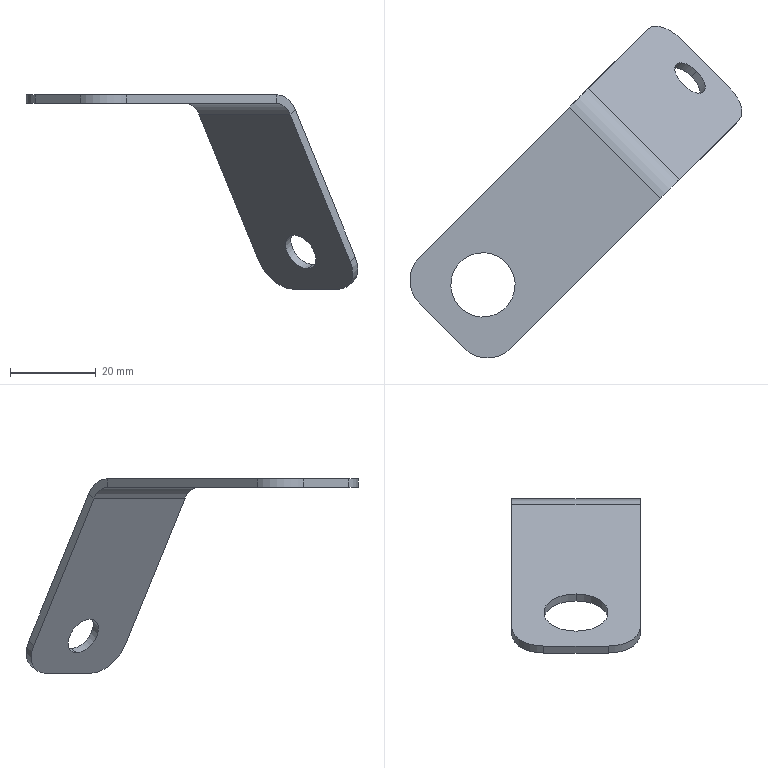Component | SolidWorks | LiftingRing(No.36)-1 | 1 solid | 22 faces | box 77.41 x 77.41 x 45.3 mm | volume 6053 mm3 | plane 12 | cylinder 10 | commonest cylinder face diameters 15 x6 9 x2 10 x1 14 x1 | material Plain Carbon Steel
STEP:
#1=COLOUR_RGB('',0.7922,0.8196,0.9333);
#2=FILL_AREA_STYLE_COLOUR('',#1);
#3=FILL_AREA_STYLE('',(#2));
#4=SURFACE_STYLE_FILL_AREA(#3);
#5=SURFACE_SIDE_STYLE('',(#4));
#6=SURFACE_STYLE_USAGE(.BOTH.,#5);
#7=PRESENTATION_STYLE_ASSIGNMENT((#6));
#8=CARTESIAN_POINT('',(-11.991,-11.991,-87.982));
#9=VERTEX_POINT('',#8);
#10=CARTESIAN_POINT('',(-11.866,-11.866,-88.289));
#11=VERTEX_POINT('',#10);
#12=CARTESIAN_POINT('',(-11.928,-11.928,-88.135));
#13=DIRECTION('',(0.6124,0.6124,0.5));
#14=DIRECTION('',(0.3536,0.3536,-0.866));
#15=AXIS2_PLACEMENT_3D('',#12,#13,#14);
#16=CIRCLE('',#15,0.1772);
#17=EDGE_CURVE('',#9,#11,#16,.T.);
#18=ORIENTED_EDGE('',*,*,#17,.F.);
#19=CARTESIAN_POINT('',(-11.943,-11.943,-87.943));
#20=VERTEX_POINT('',#19);
#21=CARTESIAN_POINT('',(-11.991,-11.991,-87.982));
#22=DIRECTION('',(0.6124,0.6124,0.5));
#23=VECTOR('',#22,39.37);
#24=LINE('',#21,#23);
#25=EDGE_CURVE('',#9,#20,#24,.T.);
#26=ORIENTED_EDGE('',*,*,#25,.T.);
#27=CARTESIAN_POINT('',(-11.817,-11.817,-88.25));
#28=VERTEX_POINT('',#27);
#29=CARTESIAN_POINT('',(-11.88,-11.88,-88.096));
#30=DIRECTION('',(0.6124,0.6124,0.5));
#31=DIRECTION('',(0.3536,0.3536,-0.866));
#32=AXIS2_PLACEMENT_3D('',#29,#30,#31);
#33=CIRCLE('',#32,0.1772);
#34=EDGE_CURVE('',#20,#28,#33,.T.);
#35=ORIENTED_EDGE('',*,*,#34,.T.);
#36=CARTESIAN_POINT('',(-11.866,-11.866,-88.289));
#37=DIRECTION('',(0.6124,0.6124,0.5));
#38=VECTOR('',#37,39.37);
#39=LINE('',#36,#38);
#40=EDGE_CURVE('',#11,#28,#39,.T.);
#41=ORIENTED_EDGE('',*,*,#40,.F.);
#42=EDGE_LOOP('',(#18,#26,#35,#41));
#43=FACE_OUTER_BOUND('',#42,.T.);
#44=CARTESIAN_POINT('',(-11.928,-11.928,-88.135));
#45=DIRECTION('',(0.6124,0.6124,0.5));
#46=DIRECTION('',(0.3536,0.3536,-0.866));
#47=AXIS2_PLACEMENT_3D('',#44,#45,#46);
#48=CYLINDRICAL_SURFACE('',#47,0.1772);
#49=ADVANCED_FACE('',(#43),#48,.F.);
#50=CARTESIAN_POINT('',(-13.988,-13.988,-86.772));
#51=VERTEX_POINT('',#50);
#52=CARTESIAN_POINT('',(-13.571,-13.571,-86.772));
#53=VERTEX_POINT('',#52);
#54=CARTESIAN_POINT('',(-13.78,-13.78,-86.772));
#55=DIRECTION('',(0.,-0.,1.));
#56=DIRECTION('',(0.7071,0.7071,0.));
#57=AXIS2_PLACEMENT_3D('',#54,#55,#56);
#58=CIRCLE('',#57,0.2953);
#59=EDGE_CURVE('',#51,#53,#58,.T.);
#60=ORIENTED_EDGE('',*,*,#59,.F.);
#61=CARTESIAN_POINT('',(-13.988,-13.988,-86.693));
#62=VERTEX_POINT('',#61);
#63=CARTESIAN_POINT('',(-13.988,-13.988,-86.772));
#64=DIRECTION('',(0.,-0.,1.));
#65=VECTOR('',#64,39.37);
#66=LINE('',#63,#65);
#67=EDGE_CURVE('',#51,#62,#66,.T.);
#68=ORIENTED_EDGE('',*,*,#67,.T.);
#69=CARTESIAN_POINT('',(-13.571,-13.571,-86.693));
#70=VERTEX_POINT('',#69);
#71=CARTESIAN_POINT('',(-13.78,-13.78,-86.693));
#72=DIRECTION('',(0.,-0.,1.));
#73=DIRECTION('',(0.7071,0.7071,0.));
#74=AXIS2_PLACEMENT_3D('',#71,#72,#73);
#75=CIRCLE('',#74,0.2953);
#76=EDGE_CURVE('',#62,#70,#75,.T.);
#77=ORIENTED_EDGE('',*,*,#76,.T.);
#78=CARTESIAN_POINT('',(-13.571,-13.571,-86.772));
#79=DIRECTION('',(0.,-0.,1.));
#80=VECTOR('',#79,39.37);
#81=LINE('',#78,#80);
#82=EDGE_CURVE('',#53,#70,#81,.T.);
#83=ORIENTED_EDGE('',*,*,#82,.F.);
#84=EDGE_LOOP('',(#60,#68,#77,#83));
#85=FACE_OUTER_BOUND('',#84,.T.);
#86=CARTESIAN_POINT('',(-13.78,-13.78,-86.772));
#87=DIRECTION('',(0.,-0.,1.));
#88=DIRECTION('',(0.7071,0.7071,0.));
#89=AXIS2_PLACEMENT_3D('',#86,#87,#88);
#90=CYLINDRICAL_SURFACE('',#89,0.2953);
#91=ADVANCED_FACE('',(#85),#90,.F.);
#92=CARTESIAN_POINT('',(-12.862,-12.027,-86.87));
#93=VERTEX_POINT('',#92);
#94=CARTESIAN_POINT('',(-12.814,-11.979,-86.831));
#95=VERTEX_POINT('',#94);
#96=CARTESIAN_POINT('',(-12.862,-12.027,-86.87));
#97=DIRECTION('',(0.6124,0.6124,0.5));
#98=VECTOR('',#97,39.37);
#99=LINE('',#96,#98);
#100=EDGE_CURVE('',#93,#95,#99,.T.);
#101=ORIENTED_EDGE('',*,*,#100,.F.);
#102=CARTESIAN_POINT('',(-12.983,-12.148,-86.772));
#103=VERTEX_POINT('',#102);
#104=CARTESIAN_POINT('',(-12.983,-12.148,-86.969));
#105=DIRECTION('',(-0.7071,0.7071,0.));
#106=DIRECTION('',(0.,0.,1.));
#107=AXIS2_PLACEMENT_3D('',#104,#105,#106);
#108=CIRCLE('',#107,0.1969);
#109=EDGE_CURVE('',#103,#93,#108,.T.);
#110=ORIENTED_EDGE('',*,*,#109,.F.);
#111=CARTESIAN_POINT('',(-12.983,-12.148,-86.693));
#112=VERTEX_POINT('',#111);
#113=CARTESIAN_POINT('',(-12.983,-12.148,-86.693));
#114=DIRECTION('',(-0.,0.,-1.));
#115=VECTOR('',#114,39.37);
#116=LINE('',#113,#115);
#117=EDGE_CURVE('',#112,#103,#116,.T.);
#118=ORIENTED_EDGE('',*,*,#117,.F.);
#119=CARTESIAN_POINT('',(-12.983,-12.148,-86.969));
#120=DIRECTION('',(-0.7071,0.7071,0.));
#121=DIRECTION('',(0.,0.,-1.));
#122=AXIS2_PLACEMENT_3D('',#119,#120,#121);
#123=CIRCLE('',#122,0.2756);
#124=EDGE_CURVE('',#112,#95,#123,.T.);
#125=ORIENTED_EDGE('',*,*,#124,.T.);
#126=EDGE_LOOP('',(#101,#110,#118,#125));
#127=FACE_OUTER_BOUND('',#126,.T.);
#128=CARTESIAN_POINT('',(-12.862,-12.027,-86.87));
#129=DIRECTION('',(-0.7071,0.7071,0.));
#130=DIRECTION('',(-0.,0.,-1.));
#131=AXIS2_PLACEMENT_3D('',#128,#129,#130);
#132=PLANE('',#131);
#133=ADVANCED_FACE('',(#127),#132,.T.);
#134=CARTESIAN_POINT('',(-12.263,-11.428,-88.181));
#135=VERTEX_POINT('',#134);
#136=CARTESIAN_POINT('',(-12.854,-12.019,-86.732));
#137=DIRECTION('',(0.3536,0.3536,-0.866));
#138=VECTOR('',#137,39.37);
#139=LINE('',#136,#138);
#140=EDGE_CURVE('',#95,#135,#139,.T.);
#141=ORIENTED_EDGE('',*,*,#140,.T.);
#142=CARTESIAN_POINT('',(-12.311,-11.476,-88.221));
#143=VERTEX_POINT('',#142);
#144=CARTESIAN_POINT('',(-12.347,-11.512,-88.25));
#145=DIRECTION('',(-0.6124,-0.6124,-0.5));
#146=VECTOR('',#145,39.37);
#147=LINE('',#144,#146);
#148=EDGE_CURVE('',#135,#143,#147,.T.);
#149=ORIENTED_EDGE('',*,*,#148,.T.);
#150=CARTESIAN_POINT('',(-12.903,-12.067,-86.772));
#151=DIRECTION('',(0.3536,0.3536,-0.866));
#152=VECTOR('',#151,39.37);
#153=LINE('',#150,#152);
#154=EDGE_CURVE('',#93,#143,#153,.T.);
#155=ORIENTED_EDGE('',*,*,#154,.F.);
#156=ORIENTED_EDGE('',*,*,#100,.T.);
#157=EDGE_LOOP('',(#141,#149,#155,#156));
#158=FACE_OUTER_BOUND('',#157,.T.);
#159=CARTESIAN_POINT('',(-12.983,-12.148,-86.693));
#160=DIRECTION('',(-0.7071,0.7071,0.));
#161=DIRECTION('',(-0.,0.,-1.));
#162=AXIS2_PLACEMENT_3D('',#159,#160,#161);
#163=PLANE('',#162);
#164=ADVANCED_FACE('',(#158),#163,.T.);
#165=CARTESIAN_POINT('',(-12.148,-12.983,-86.772));
#166=VERTEX_POINT('',#165);
#167=CARTESIAN_POINT('',(-12.148,-12.983,-86.693));
#168=VERTEX_POINT('',#167);
#169=CARTESIAN_POINT('',(-12.148,-12.983,-86.772));
#170=DIRECTION('',(0.,-0.,1.));
#171=VECTOR('',#170,39.37);
#172=LINE('',#169,#171);
#173=EDGE_CURVE('',#166,#168,#172,.T.);
#174=ORIENTED_EDGE('',*,*,#173,.F.);
#175=CARTESIAN_POINT('',(-12.027,-12.862,-86.87));
#176=VERTEX_POINT('',#175);
#177=CARTESIAN_POINT('',(-12.148,-12.983,-86.969));
#178=DIRECTION('',(-0.7071,0.7071,0.));
#179=DIRECTION('',(0.,0.,1.));
#180=AXIS2_PLACEMENT_3D('',#177,#178,#179);
#181=CIRCLE('',#180,0.1969);
#182=EDGE_CURVE('',#166,#176,#181,.T.);
#183=ORIENTED_EDGE('',*,*,#182,.T.);
#184=CARTESIAN_POINT('',(-11.979,-12.814,-86.831));
#185=VERTEX_POINT('',#184);
#186=CARTESIAN_POINT('',(-11.979,-12.814,-86.831));
#187=DIRECTION('',(-0.6124,-0.6124,-0.5));
#188=VECTOR('',#187,39.37);
#189=LINE('',#186,#188);
#190=EDGE_CURVE('',#185,#176,#189,.T.);
#191=ORIENTED_EDGE('',*,*,#190,.F.);
#192=CARTESIAN_POINT('',(-12.148,-12.983,-86.969));
#193=DIRECTION('',(-0.7071,0.7071,0.));
#194=DIRECTION('',(0.,0.,-1.));
#195=AXIS2_PLACEMENT_3D('',#192,#193,#194);
#196=CIRCLE('',#195,0.2756);
#197=EDGE_CURVE('',#168,#185,#196,.T.);
#198=ORIENTED_EDGE('',*,*,#197,.F.);
#199=EDGE_LOOP('',(#174,#183,#191,#198));
#200=FACE_OUTER_BOUND('',#199,.T.);
#201=CARTESIAN_POINT('',(-12.148,-12.983,-86.772));
#202=DIRECTION('',(0.7071,-0.7071,-0.));
#203=DIRECTION('',(0.,-0.,1.));
#204=AXIS2_PLACEMENT_3D('',#201,#202,#203);
#205=PLANE('',#204);
#206=ADVANCED_FACE('',(#200),#205,.T.);
#207=CARTESIAN_POINT('',(-13.529,-14.364,-86.693));
#208=VERTEX_POINT('',#207);
#209=CARTESIAN_POINT('',(-13.738,-14.573,-86.693));
#210=DIRECTION('',(0.7071,0.7071,-0.));
#211=VECTOR('',#210,39.37);
#212=LINE('',#209,#211);
#213=EDGE_CURVE('',#208,#168,#212,.T.);
#214=ORIENTED_EDGE('',*,*,#213,.F.);
#215=CARTESIAN_POINT('',(-13.529,-14.364,-86.772));
#216=VERTEX_POINT('',#215);
#217=CARTESIAN_POINT('',(-13.529,-14.364,-86.831));
#218=DIRECTION('',(-0.,0.,-1.));
#219=VECTOR('',#218,39.37);
#220=LINE('',#217,#219);
#221=EDGE_CURVE('',#208,#216,#220,.T.);
#222=ORIENTED_EDGE('',*,*,#221,.T.);
#223=CARTESIAN_POINT('',(-13.738,-14.573,-86.772));
#224=DIRECTION('',(0.7071,0.7071,-0.));
#225=VECTOR('',#224,39.37);
#226=LINE('',#223,#225);
#227=EDGE_CURVE('',#216,#166,#226,.T.);
#228=ORIENTED_EDGE('',*,*,#227,.T.);
#229=ORIENTED_EDGE('',*,*,#173,.T.);
#230=EDGE_LOOP('',(#214,#222,#228,#229));
#231=FACE_OUTER_BOUND('',#230,.T.);
#232=CARTESIAN_POINT('',(-11.979,-12.814,-86.831));
#233=DIRECTION('',(0.7071,-0.7071,-0.));
#234=DIRECTION('',(0.,-0.,1.));
#235=AXIS2_PLACEMENT_3D('',#232,#233,#234);
#236=PLANE('',#235);
#237=ADVANCED_FACE('',(#231),#236,.T.);
#238=CARTESIAN_POINT('',(-11.88,-11.88,-88.096));
#239=DIRECTION('',(0.6124,0.6124,0.5));
#240=DIRECTION('',(0.3536,0.3536,-0.866));
#241=AXIS2_PLACEMENT_3D('',#238,#239,#240);
#242=CIRCLE('',#241,0.1772);
#243=EDGE_CURVE('',#28,#20,#242,.T.);
#244=ORIENTED_EDGE('',*,*,#243,.F.);
#245=ORIENTED_EDGE('',*,*,#34,.F.);
#246=EDGE_LOOP('',(#244,#245));
#247=FACE_BOUND('',#246,.T.);
#248=CARTESIAN_POINT('',(-11.95,-11.532,-88.437));
#249=VERTEX_POINT('',#248);
#250=CARTESIAN_POINT('',(-11.532,-11.95,-88.437));
#251=VERTEX_POINT('',#250);
#252=CARTESIAN_POINT('',(-12.158,-11.323,-88.437));
#253=DIRECTION('',(0.7071,-0.7071,-0.));
#254=VECTOR('',#253,39.37);
#255=LINE('',#252,#254);
#256=EDGE_CURVE('',#249,#251,#255,.T.);
#257=ORIENTED_EDGE('',*,*,#256,.F.);
#258=CARTESIAN_POINT('',(-12.054,-11.636,-88.181));
#259=DIRECTION('',(0.6124,0.6124,0.5));
#260=DIRECTION('',(-0.3536,-0.3536,0.866));
#261=AXIS2_PLACEMENT_3D('',#258,#259,#260);
#262=CIRCLE('',#261,0.2953);
#263=EDGE_CURVE('',#249,#135,#262,.T.);
#264=ORIENTED_EDGE('',*,*,#263,.T.);
#265=ORIENTED_EDGE('',*,*,#140,.F.);
#266=CARTESIAN_POINT('',(-12.814,-11.979,-86.831));
#267=DIRECTION('',(0.7071,-0.7071,-0.));
#268=VECTOR('',#267,39.37);
#269=LINE('',#266,#268);
#270=EDGE_CURVE('',#95,#185,#269,.T.);
#271=ORIENTED_EDGE('',*,*,#270,.T.);
#272=CARTESIAN_POINT('',(-11.428,-12.263,-88.181));
#273=VERTEX_POINT('',#272);
#274=CARTESIAN_POINT('',(-12.019,-12.854,-86.732));
#275=DIRECTION('',(0.3536,0.3536,-0.866));
#276=VECTOR('',#275,39.37);
#277=LINE('',#274,#276);
#278=EDGE_CURVE('',#185,#273,#277,.T.);
#279=ORIENTED_EDGE('',*,*,#278,.T.);
#280=CARTESIAN_POINT('',(-11.636,-12.054,-88.181));
#281=DIRECTION('',(0.6124,0.6124,0.5));
#282=DIRECTION('',(-0.3536,-0.3536,0.866));
#283=AXIS2_PLACEMENT_3D('',#280,#281,#282);
#284=CIRCLE('',#283,0.2953);
#285=EDGE_CURVE('',#273,#251,#284,.T.);
#286=ORIENTED_EDGE('',*,*,#285,.T.);
#287=EDGE_LOOP('',(#257,#264,#265,#271,#279,#286));
#288=FACE_OUTER_BOUND('',#287,.T.);
#289=CARTESIAN_POINT('',(-12.854,-12.019,-86.732));
#290=DIRECTION('',(-0.6124,-0.6124,-0.5));
#291=DIRECTION('',(-0.3536,-0.3536,0.866));
#292=AXIS2_PLACEMENT_3D('',#289,#290,#291);
#293=PLANE('',#292);
#294=ADVANCED_FACE('',(#247,#288),#293,.F.);
#295=CARTESIAN_POINT('',(-11.998,-11.58,-88.476));
#296=VERTEX_POINT('',#295);
#297=CARTESIAN_POINT('',(-11.58,-11.998,-88.476));
#298=VERTEX_POINT('',#297);
#299=CARTESIAN_POINT('',(-12.207,-11.371,-88.476));
#300=DIRECTION('',(0.7071,-0.7071,-0.));
#301=VECTOR('',#300,39.37);
#302=LINE('',#299,#301);
#303=EDGE_CURVE('',#296,#298,#302,.T.);
#304=ORIENTED_EDGE('',*,*,#303,.F.);
#305=CARTESIAN_POINT('',(-11.998,-11.58,-88.476));
#306=DIRECTION('',(0.6124,0.6124,0.5));
#307=VECTOR('',#306,39.37);
#308=LINE('',#305,#307);
#309=EDGE_CURVE('',#296,#249,#308,.T.);
#310=ORIENTED_EDGE('',*,*,#309,.T.);
#311=ORIENTED_EDGE('',*,*,#256,.T.);
#312=CARTESIAN_POINT('',(-11.58,-11.998,-88.476));
#313=DIRECTION('',(-0.6124,-0.6124,-0.5));
#314=VECTOR('',#313,39.37);
#315=LINE('',#312,#314);
#316=EDGE_CURVE('',#251,#298,#315,.T.);
#317=ORIENTED_EDGE('',*,*,#316,.T.);
#318=EDGE_LOOP('',(#304,#310,#311,#317));
#319=FACE_OUTER_BOUND('',#318,.T.);
#320=CARTESIAN_POINT('',(-12.207,-11.371,-88.476));
#321=DIRECTION('',(0.3536,0.3536,-0.866));
#322=DIRECTION('',(-0.6124,-0.6124,-0.5));
#323=AXIS2_PLACEMENT_3D('',#320,#321,#322);
#324=PLANE('',#323);
#325=ADVANCED_FACE('',(#319),#324,.T.);
#326=CARTESIAN_POINT('',(-11.928,-11.928,-88.135));
#327=DIRECTION('',(0.6124,0.6124,0.5));
#328=DIRECTION('',(0.3536,0.3536,-0.866));
#329=AXIS2_PLACEMENT_3D('',#326,#327,#328);
#330=CIRCLE('',#329,0.1772);
#331=EDGE_CURVE('',#11,#9,#330,.T.);
#332=ORIENTED_EDGE('',*,*,#331,.T.);
#333=ORIENTED_EDGE('',*,*,#17,.T.);
#334=EDGE_LOOP('',(#332,#333));
#335=FACE_BOUND('',#334,.T.);
#336=ORIENTED_EDGE('',*,*,#154,.T.);
#337=CARTESIAN_POINT('',(-12.102,-11.685,-88.221));
#338=DIRECTION('',(-0.6124,-0.6124,-0.5));
#339=DIRECTION('',(-0.3536,-0.3536,0.866));
#340=AXIS2_PLACEMENT_3D('',#337,#338,#339);
#341=CIRCLE('',#340,0.2953);
#342=EDGE_CURVE('',#143,#296,#341,.T.);
#343=ORIENTED_EDGE('',*,*,#342,.T.);
#344=ORIENTED_EDGE('',*,*,#303,.T.);
#345=CARTESIAN_POINT('',(-11.476,-12.311,-88.221));
#346=VERTEX_POINT('',#345);
#347=CARTESIAN_POINT('',(-11.685,-12.102,-88.221));
#348=DIRECTION('',(-0.6124,-0.6124,-0.5));
#349=DIRECTION('',(-0.3536,-0.3536,0.866));
#350=AXIS2_PLACEMENT_3D('',#347,#348,#349);
#351=CIRCLE('',#350,0.2953);
#352=EDGE_CURVE('',#298,#346,#351,.T.);
#353=ORIENTED_EDGE('',*,*,#352,.T.);
#354=CARTESIAN_POINT('',(-12.067,-12.903,-86.772));
#355=DIRECTION('',(0.3536,0.3536,-0.866));
#356=VECTOR('',#355,39.37);
#357=LINE('',#354,#356);
#358=EDGE_CURVE('',#176,#346,#357,.T.);
#359=ORIENTED_EDGE('',*,*,#358,.F.);
#360=CARTESIAN_POINT('',(-12.862,-12.027,-86.87));
#361=DIRECTION('',(0.7071,-0.7071,-0.));
#362=VECTOR('',#361,39.37);
#363=LINE('',#360,#362);
#364=EDGE_CURVE('',#93,#176,#363,.T.);
#365=ORIENTED_EDGE('',*,*,#364,.F.);
#366=EDGE_LOOP('',(#336,#343,#344,#353,#359,#365));
#367=FACE_OUTER_BOUND('',#366,.T.);
#368=CARTESIAN_POINT('',(-12.903,-12.067,-86.772));
#369=DIRECTION('',(-0.6124,-0.6124,-0.5));
#370=DIRECTION('',(-0.3536,-0.3536,0.866));
#371=AXIS2_PLACEMENT_3D('',#368,#369,#370);
#372=PLANE('',#371);
#373=ADVANCED_FACE('',(#335,#367),#372,.T.);
#374=ORIENTED_EDGE('',*,*,#182,.F.);
#375=CARTESIAN_POINT('',(-12.983,-12.148,-86.772));
#376=DIRECTION('',(0.7071,-0.7071,-0.));
#377=VECTOR('',#376,39.37);
#378=LINE('',#375,#377);
#379=EDGE_CURVE('',#103,#166,#378,.T.);
#380=ORIENTED_EDGE('',*,*,#379,.F.);
#381=ORIENTED_EDGE('',*,*,#109,.T.);
#382=ORIENTED_EDGE('',*,*,#364,.T.);
#383=EDGE_LOOP('',(#374,#380,#381,#382));
#384=FACE_OUTER_BOUND('',#383,.T.);
#385=CARTESIAN_POINT('',(-12.983,-12.148,-86.969));
#386=DIRECTION('',(0.7071,-0.7071,-0.));
#387=DIRECTION('',(0.,0.,1.));
#388=AXIS2_PLACEMENT_3D('',#385,#386,#387);
#389=CYLINDRICAL_SURFACE('',#388,0.1969);
#390=ADVANCED_FACE('',(#384),#389,.F.);
#391=CARTESIAN_POINT('',(-13.78,-13.78,-86.772));
#392=DIRECTION('',(0.,-0.,1.));
#393=DIRECTION('',(0.7071,0.7071,0.));
#394=AXIS2_PLACEMENT_3D('',#391,#392,#393);
#395=CIRCLE('',#394,0.2953);
#396=EDGE_CURVE('',#53,#51,#395,.T.);
#397=ORIENTED_EDGE('',*,*,#396,.T.);
#398=ORIENTED_EDGE('',*,*,#59,.T.);
#399=EDGE_LOOP('',(#397,#398));
#400=FACE_BOUND('',#399,.T.);
#401=ORIENTED_EDGE('',*,*,#227,.F.);
#402=CARTESIAN_POINT('',(-13.947,-14.364,-86.772));
#403=VERTEX_POINT('',#402);
#404=CARTESIAN_POINT('',(-13.738,-14.155,-86.772));
#405=DIRECTION('',(-0.,0.,-1.));
#406=DIRECTION('',(-0.7071,-0.7071,0.));
#407=AXIS2_PLACEMENT_3D('',#404,#405,#406);
#408=CIRCLE('',#407,0.2953);
#409=EDGE_CURVE('',#216,#403,#408,.T.);
#410=ORIENTED_EDGE('',*,*,#409,.T.);
#411=CARTESIAN_POINT('',(-14.364,-13.947,-86.772));
#412=VERTEX_POINT('',#411);
#413=CARTESIAN_POINT('',(-14.573,-13.738,-86.772));
#414=DIRECTION('',(0.7071,-0.7071,-0.));
#415=VECTOR('',#414,39.37);
#416=LINE('',#413,#415);
#417=EDGE_CURVE('',#412,#403,#416,.T.);
#418=ORIENTED_EDGE('',*,*,#417,.F.);
#419=CARTESIAN_POINT('',(-14.364,-13.529,-86.772));
#420=VERTEX_POINT('',#419);
#421=CARTESIAN_POINT('',(-14.155,-13.738,-86.772));
#422=DIRECTION('',(-0.,0.,-1.));
#423=DIRECTION('',(-0.7071,-0.7071,0.));
#424=AXIS2_PLACEMENT_3D('',#421,#422,#423);
#425=CIRCLE('',#424,0.2953);
#426=EDGE_CURVE('',#412,#420,#425,.T.);
#427=ORIENTED_EDGE('',*,*,#426,.T.);
#428=CARTESIAN_POINT('',(-14.573,-13.738,-86.772));
#429=DIRECTION('',(0.7071,0.7071,-0.));
#430=VECTOR('',#429,39.37);
#431=LINE('',#428,#430);
#432=EDGE_CURVE('',#420,#103,#431,.T.);
#433=ORIENTED_EDGE('',*,*,#432,.T.);
#434=ORIENTED_EDGE('',*,*,#379,.T.);
#435=EDGE_LOOP('',(#401,#410,#418,#427,#433,#434));
#436=FACE_OUTER_BOUND('',#435,.T.);
#437=CARTESIAN_POINT('',(-14.573,-13.738,-86.772));
#438=DIRECTION('',(-0.,0.,-1.));
#439=DIRECTION('',(-0.7071,-0.7071,0.));
#440=AXIS2_PLACEMENT_3D('',#437,#438,#439);
#441=PLANE('',#440);
#442=ADVANCED_FACE('',(#400,#436),#441,.T.);
#443=ORIENTED_EDGE('',*,*,#417,.T.);
#444=CARTESIAN_POINT('',(-13.947,-14.364,-86.693));
#445=VERTEX_POINT('',#444);
#446=CARTESIAN_POINT('',(-13.947,-14.364,-86.693));
#447=DIRECTION('',(0.,-0.,1.));
#448=VECTOR('',#447,39.37);
#449=LINE('',#446,#448);
#450=EDGE_CURVE('',#403,#445,#449,.T.);
#451=ORIENTED_EDGE('',*,*,#450,.T.);
#452=CARTESIAN_POINT('',(-14.364,-13.947,-86.693));
#453=VERTEX_POINT('',#452);
#454=CARTESIAN_POINT('',(-14.573,-13.738,-86.693));
#455=DIRECTION('',(0.7071,-0.7071,-0.));
#456=VECTOR('',#455,39.37);
#457=LINE('',#454,#456);
#458=EDGE_CURVE('',#453,#445,#457,.T.);
#459=ORIENTED_EDGE('',*,*,#458,.F.);
#460=CARTESIAN_POINT('',(-14.364,-13.947,-86.772));
#461=DIRECTION('',(-0.,0.,-1.));
#462=VECTOR('',#461,39.37);
#463=LINE('',#460,#462);
#464=EDGE_CURVE('',#453,#412,#463,.T.);
#465=ORIENTED_EDGE('',*,*,#464,.T.);
#466=EDGE_LOOP('',(#443,#451,#459,#465));
#467=FACE_OUTER_BOUND('',#466,.T.);
#468=CARTESIAN_POINT('',(-14.573,-13.738,-86.693));
#469=DIRECTION('',(-0.7071,-0.7071,0.));
#470=DIRECTION('',(-0.7071,0.7071,0.));
#471=AXIS2_PLACEMENT_3D('',#468,#469,#470);
#472=PLANE('',#471);
#473=ADVANCED_FACE('',(#467),#472,.T.);
#474=CARTESIAN_POINT('',(-13.78,-13.78,-86.693));
#475=DIRECTION('',(0.,-0.,1.));
#476=DIRECTION('',(0.7071,0.7071,0.));
#477=AXIS2_PLACEMENT_3D('',#474,#475,#476);
#478=CIRCLE('',#477,0.2953);
#479=EDGE_CURVE('',#70,#62,#478,.T.);
#480=ORIENTED_EDGE('',*,*,#479,.F.);
#481=ORIENTED_EDGE('',*,*,#76,.F.);
#482=EDGE_LOOP('',(#480,#481));
#483=FACE_BOUND('',#482,.T.);
#484=ORIENTED_EDGE('',*,*,#458,.T.);
#485=CARTESIAN_POINT('',(-13.738,-14.155,-86.693));
#486=DIRECTION('',(0.,-0.,1.));
#487=DIRECTION('',(-0.7071,-0.7071,0.));
#488=AXIS2_PLACEMENT_3D('',#485,#486,#487);
#489=CIRCLE('',#488,0.2953);
#490=EDGE_CURVE('',#445,#208,#489,.T.);
#491=ORIENTED_EDGE('',*,*,#490,.T.);
#492=ORIENTED_EDGE('',*,*,#213,.T.);
#493=CARTESIAN_POINT('',(-12.983,-12.148,-86.693));
#494=DIRECTION('',(0.7071,-0.7071,-0.));
#495=VECTOR('',#494,39.37);
#496=LINE('',#493,#495);
#497=EDGE_CURVE('',#112,#168,#496,.T.);
#498=ORIENTED_EDGE('',*,*,#497,.F.);
#499=CARTESIAN_POINT('',(-14.364,-13.529,-86.693));
#500=VERTEX_POINT('',#499);
#501=CARTESIAN_POINT('',(-14.573,-13.738,-86.693));
#502=DIRECTION('',(0.7071,0.7071,-0.));
#503=VECTOR('',#502,39.37);
#504=LINE('',#501,#503);
#505=EDGE_CURVE('',#500,#112,#504,.T.);
#506=ORIENTED_EDGE('',*,*,#505,.F.);
#507=CARTESIAN_POINT('',(-14.155,-13.738,-86.693));
#508=DIRECTION('',(0.,-0.,1.));
#509=DIRECTION('',(-0.7071,-0.7071,0.));
#510=AXIS2_PLACEMENT_3D('',#507,#508,#509);
#511=CIRCLE('',#510,0.2953);
#512=EDGE_CURVE('',#500,#453,#511,.T.);
#513=ORIENTED_EDGE('',*,*,#512,.T.);
#514=EDGE_LOOP('',(#484,#491,#492,#498,#506,#513));
#515=FACE_OUTER_BOUND('',#514,.T.);
#516=CARTESIAN_POINT('',(-14.573,-13.738,-86.693));
#517=DIRECTION('',(-0.,0.,-1.));
#518=DIRECTION('',(-0.7071,-0.7071,0.));
#519=AXIS2_PLACEMENT_3D('',#516,#517,#518);
#520=PLANE('',#519);
#521=ADVANCED_FACE('',(#483,#515),#520,.F.);
#522=ORIENTED_EDGE('',*,*,#197,.T.);
#523=ORIENTED_EDGE('',*,*,#270,.F.);
#524=ORIENTED_EDGE('',*,*,#124,.F.);
#525=ORIENTED_EDGE('',*,*,#497,.T.);
#526=EDGE_LOOP('',(#522,#523,#524,#525));
#527=FACE_OUTER_BOUND('',#526,.T.);
#528=CARTESIAN_POINT('',(-12.983,-12.148,-86.969));
#529=DIRECTION('',(0.7071,-0.7071,-0.));
#530=DIRECTION('',(0.,0.,1.));
#531=AXIS2_PLACEMENT_3D('',#528,#529,#530);
#532=CYLINDRICAL_SURFACE('',#531,0.2756);
#533=ADVANCED_FACE('',(#527),#532,.T.);
#534=ORIENTED_EDGE('',*,*,#432,.F.);
#535=CARTESIAN_POINT('',(-14.364,-13.529,-86.693));
#536=DIRECTION('',(0.,-0.,1.));
#537=VECTOR('',#536,39.37);
#538=LINE('',#535,#537);
#539=EDGE_CURVE('',#420,#500,#538,.T.);
#540=ORIENTED_EDGE('',*,*,#539,.T.);
#541=ORIENTED_EDGE('',*,*,#505,.T.);
#542=ORIENTED_EDGE('',*,*,#117,.T.);
#543=EDGE_LOOP('',(#534,#540,#541,#542));
#544=FACE_OUTER_BOUND('',#543,.T.);
#545=CARTESIAN_POINT('',(-12.983,-12.148,-86.969));
#546=DIRECTION('',(0.7071,-0.7071,-0.));
#547=DIRECTION('',(0.,-0.,1.));
#548=AXIS2_PLACEMENT_3D('',#545,#546,#547);
#549=PLANE('',#548);
#550=ADVANCED_FACE('',(#544),#549,.F.);
#551=ORIENTED_EDGE('',*,*,#358,.T.);
#552=CARTESIAN_POINT('',(-11.596,-12.432,-88.319));
#553=DIRECTION('',(0.6124,0.6124,0.5));
#554=VECTOR('',#553,39.37);
#555=LINE('',#552,#554);
#556=EDGE_CURVE('',#346,#273,#555,.T.);
#557=ORIENTED_EDGE('',*,*,#556,.T.);
#558=ORIENTED_EDGE('',*,*,#278,.F.);
#559=ORIENTED_EDGE('',*,*,#190,.T.);
#560=EDGE_LOOP('',(#551,#557,#558,#559));
#561=FACE_OUTER_BOUND('',#560,.T.);
#562=CARTESIAN_POINT('',(-12.148,-12.983,-86.969));
#563=DIRECTION('',(0.7071,-0.7071,-0.));
#564=DIRECTION('',(0.,-0.,1.));
#565=AXIS2_PLACEMENT_3D('',#562,#563,#564);
#566=PLANE('',#565);
#567=ADVANCED_FACE('',(#561),#566,.T.);
#568=ORIENTED_EDGE('',*,*,#342,.F.);
#569=ORIENTED_EDGE('',*,*,#148,.F.);
#570=ORIENTED_EDGE('',*,*,#263,.F.);
#571=ORIENTED_EDGE('',*,*,#309,.F.);
#572=EDGE_LOOP('',(#568,#569,#570,#571));
#573=FACE_OUTER_BOUND('',#572,.T.);
#574=CARTESIAN_POINT('',(-12.102,-11.685,-88.221));
#575=DIRECTION('',(0.6124,0.6124,0.5));
#576=DIRECTION('',(0.3536,0.3536,-0.866));
#577=AXIS2_PLACEMENT_3D('',#574,#575,#576);
#578=CYLINDRICAL_SURFACE('',#577,0.2953);
#579=ADVANCED_FACE('',(#573),#578,.T.);
#580=ORIENTED_EDGE('',*,*,#352,.F.);
#581=ORIENTED_EDGE('',*,*,#316,.F.);
#582=ORIENTED_EDGE('',*,*,#285,.F.);
#583=ORIENTED_EDGE('',*,*,#556,.F.);
#584=EDGE_LOOP('',(#580,#581,#582,#583));
#585=FACE_OUTER_BOUND('',#584,.T.);
#586=CARTESIAN_POINT('',(-11.805,-12.223,-88.319));
#587=DIRECTION('',(0.6124,0.6124,0.5));
#588=DIRECTION('',(0.3536,0.3536,-0.866));
#589=AXIS2_PLACEMENT_3D('',#586,#587,#588);
#590=CYLINDRICAL_SURFACE('',#589,0.2953);
#591=ADVANCED_FACE('',(#585),#590,.T.);
#592=ORIENTED_EDGE('',*,*,#490,.F.);
#593=ORIENTED_EDGE('',*,*,#450,.F.);
#594=ORIENTED_EDGE('',*,*,#409,.F.);
#595=ORIENTED_EDGE('',*,*,#221,.F.);
#596=EDGE_LOOP('',(#592,#593,#594,#595));
#597=FACE_OUTER_BOUND('',#596,.T.);
#598=CARTESIAN_POINT('',(-13.738,-14.155,-86.831));
#599=DIRECTION('',(-0.,0.,-1.));
#600=DIRECTION('',(0.7071,-0.7071,0.));
#601=AXIS2_PLACEMENT_3D('',#598,#599,#600);
#602=CYLINDRICAL_SURFACE('',#601,0.2953);
#603=ADVANCED_FACE('',(#597),#602,.T.);
#604=ORIENTED_EDGE('',*,*,#512,.F.);
#605=ORIENTED_EDGE('',*,*,#539,.F.);
#606=ORIENTED_EDGE('',*,*,#426,.F.);
#607=ORIENTED_EDGE('',*,*,#464,.F.);
#608=EDGE_LOOP('',(#604,#605,#606,#607));
#609=FACE_OUTER_BOUND('',#608,.T.);
#610=CARTESIAN_POINT('',(-14.155,-13.738,-86.693));
#611=DIRECTION('',(0.,-0.,1.));
#612=DIRECTION('',(-0.7071,0.7071,0.));
#613=AXIS2_PLACEMENT_3D('',#610,#611,#612);
#614=CYLINDRICAL_SURFACE('',#613,0.2953);
#615=ADVANCED_FACE('',(#609),#614,.T.);
#616=ORIENTED_EDGE('',*,*,#67,.F.);
#617=ORIENTED_EDGE('',*,*,#396,.F.);
#618=ORIENTED_EDGE('',*,*,#82,.T.);
#619=ORIENTED_EDGE('',*,*,#479,.T.);
#620=EDGE_LOOP('',(#616,#617,#618,#619));
#621=FACE_OUTER_BOUND('',#620,.T.);
#622=CARTESIAN_POINT('',(-13.78,-13.78,-86.772));
#623=DIRECTION('',(0.,-0.,1.));
#624=DIRECTION('',(0.7071,0.7071,0.));
#625=AXIS2_PLACEMENT_3D('',#622,#623,#624);
#626=CYLINDRICAL_SURFACE('',#625,0.2953);
#627=ADVANCED_FACE('',(#621),#626,.F.);
#628=ORIENTED_EDGE('',*,*,#25,.F.);
#629=ORIENTED_EDGE('',*,*,#331,.F.);
#630=ORIENTED_EDGE('',*,*,#40,.T.);
#631=ORIENTED_EDGE('',*,*,#243,.T.);
#632=EDGE_LOOP('',(#628,#629,#630,#631));
#633=FACE_OUTER_BOUND('',#632,.T.);
#634=CARTESIAN_POINT('',(-11.928,-11.928,-88.135));
#635=DIRECTION('',(0.6124,0.6124,0.5));
#636=DIRECTION('',(0.3536,0.3536,-0.866));
#637=AXIS2_PLACEMENT_3D('',#634,#635,#636);
#638=CYLINDRICAL_SURFACE('',#637,0.1772);
#639=ADVANCED_FACE('',(#633),#638,.F.);
#640=CLOSED_SHELL('',(#49,#91,#133,#164,#206,#237,#294,#325,#373,#390,#442,#473,#521,#533,#550,#567,#579,#591,#603,#615,#627,#639));
#641=MANIFOLD_SOLID_BREP('',#640);
#642=STYLED_ITEM('',(#7),#641);
#643=PRESENTATION_LAYER_ASSIGNMENT('','',(#642));
#644=CARTESIAN_POINT('',(0.,0.,0.));
#645=DIRECTION('',(0.,0.,1.));
#646=DIRECTION('',(1.,0.,0.));
#647=AXIS2_PLACEMENT_3D('',#644,#645,#646);
#648=(LENGTH_UNIT()NAMED_UNIT(*)SI_UNIT($,.METRE.));
#649=LENGTH_MEASURE_WITH_UNIT(LENGTH_MEASURE(0.0254),#648);
#650=DIMENSIONAL_EXPONENTS(1.,0.,0.,0.,0.,0.,0.);
#651=(CONVERSION_BASED_UNIT('',#649)LENGTH_UNIT()NAMED_UNIT(#650));
#652=UNCERTAINTY_MEASURE_WITH_UNIT(LENGTH_MEASURE(0.00001),#651,'','');
#653=(NAMED_UNIT(*)PLANE_ANGLE_UNIT()SI_UNIT($,.RADIAN.));
#654=(NAMED_UNIT(*)SI_UNIT($,.STERADIAN.)SOLID_ANGLE_UNIT());
#655=(GEOMETRIC_REPRESENTATION_CONTEXT(3)GLOBAL_UNCERTAINTY_ASSIGNED_CONTEXT((#652))GLOBAL_UNIT_ASSIGNED_CONTEXT((#651,#653,#654))REPRESENTATION_CONTEXT('',''));
#656=ADVANCED_BREP_SHAPE_REPRESENTATION('',(#641,#647),#655);
#657=(LENGTH_UNIT()NAMED_UNIT(*)SI_UNIT($,.METRE.));
#658=LENGTH_MEASURE_WITH_UNIT(LENGTH_MEASURE(0.0254),#657);
#659=DIMENSIONAL_EXPONENTS(1.,0.,0.,0.,0.,0.,0.);
#660=(CONVERSION_BASED_UNIT('',#658)LENGTH_UNIT()NAMED_UNIT(#659));
#661=UNCERTAINTY_MEASURE_WITH_UNIT(LENGTH_MEASURE(0.00001),#660,'','');
#662=(NAMED_UNIT(*)PLANE_ANGLE_UNIT()SI_UNIT($,.RADIAN.));
#663=(NAMED_UNIT(*)SI_UNIT($,.STERADIAN.)SOLID_ANGLE_UNIT());
#664=(GEOMETRIC_REPRESENTATION_CONTEXT(3)GLOBAL_UNCERTAINTY_ASSIGNED_CONTEXT((#661))GLOBAL_UNIT_ASSIGNED_CONTEXT((#660,#662,#663))REPRESENTATION_CONTEXT('',''));
#665=MECHANICAL_DESIGN_GEOMETRIC_PRESENTATION_REPRESENTATION('',(#642),#664);